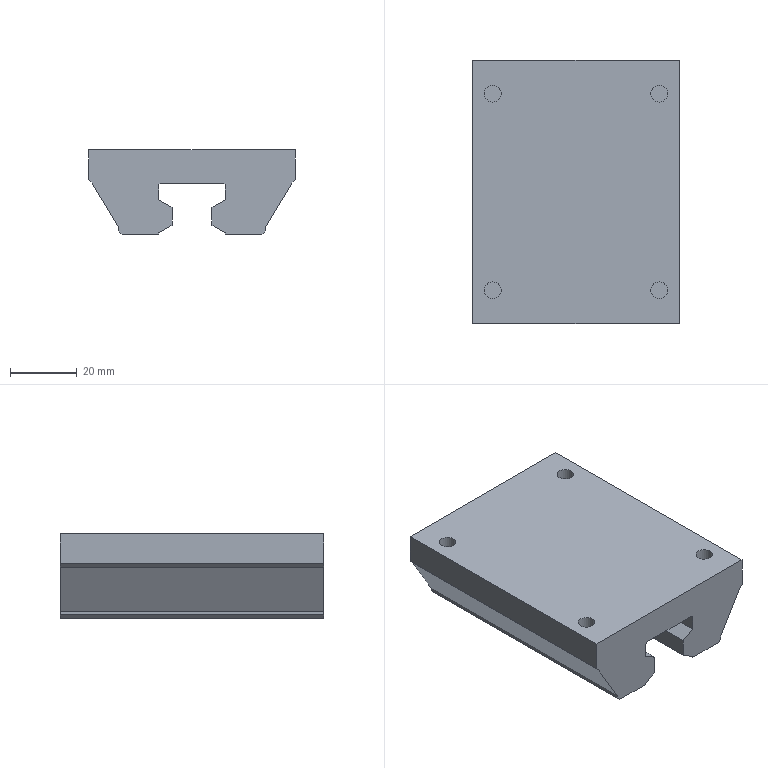Component | NX | LINEAR_SLIDER_2 | 1 solid | 36 faces | volume 90348 mm3 | plane 32 | cylinder 4 | commonest cylinder face diameters 5 x4